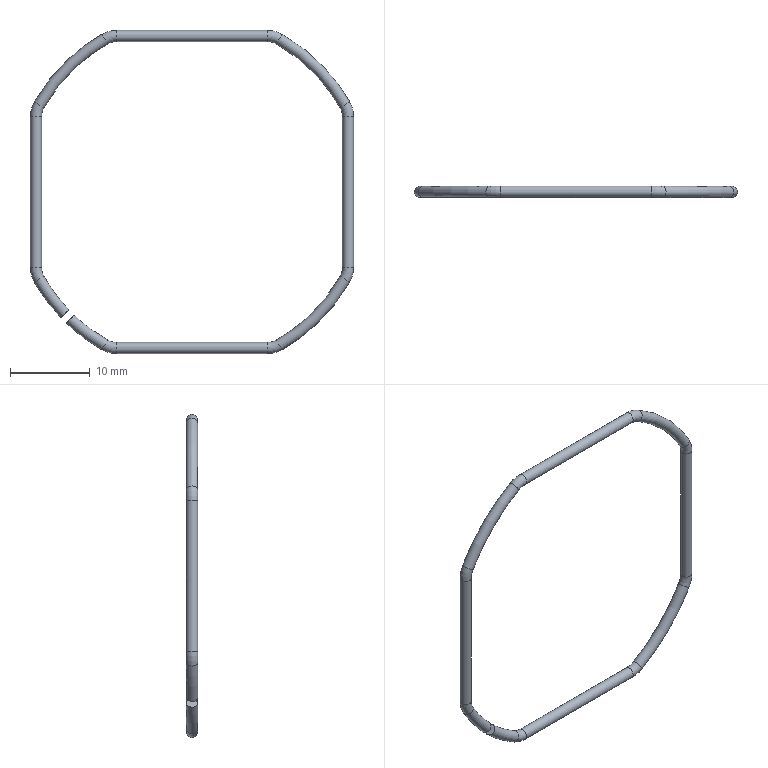Component | NX | STEEL_WIRE | 1 solid | 19 faces | volume 206 mm3 | torus 13 | cylinder 4 | plane 2 | commonest cylinder face diameters 1.4 x4